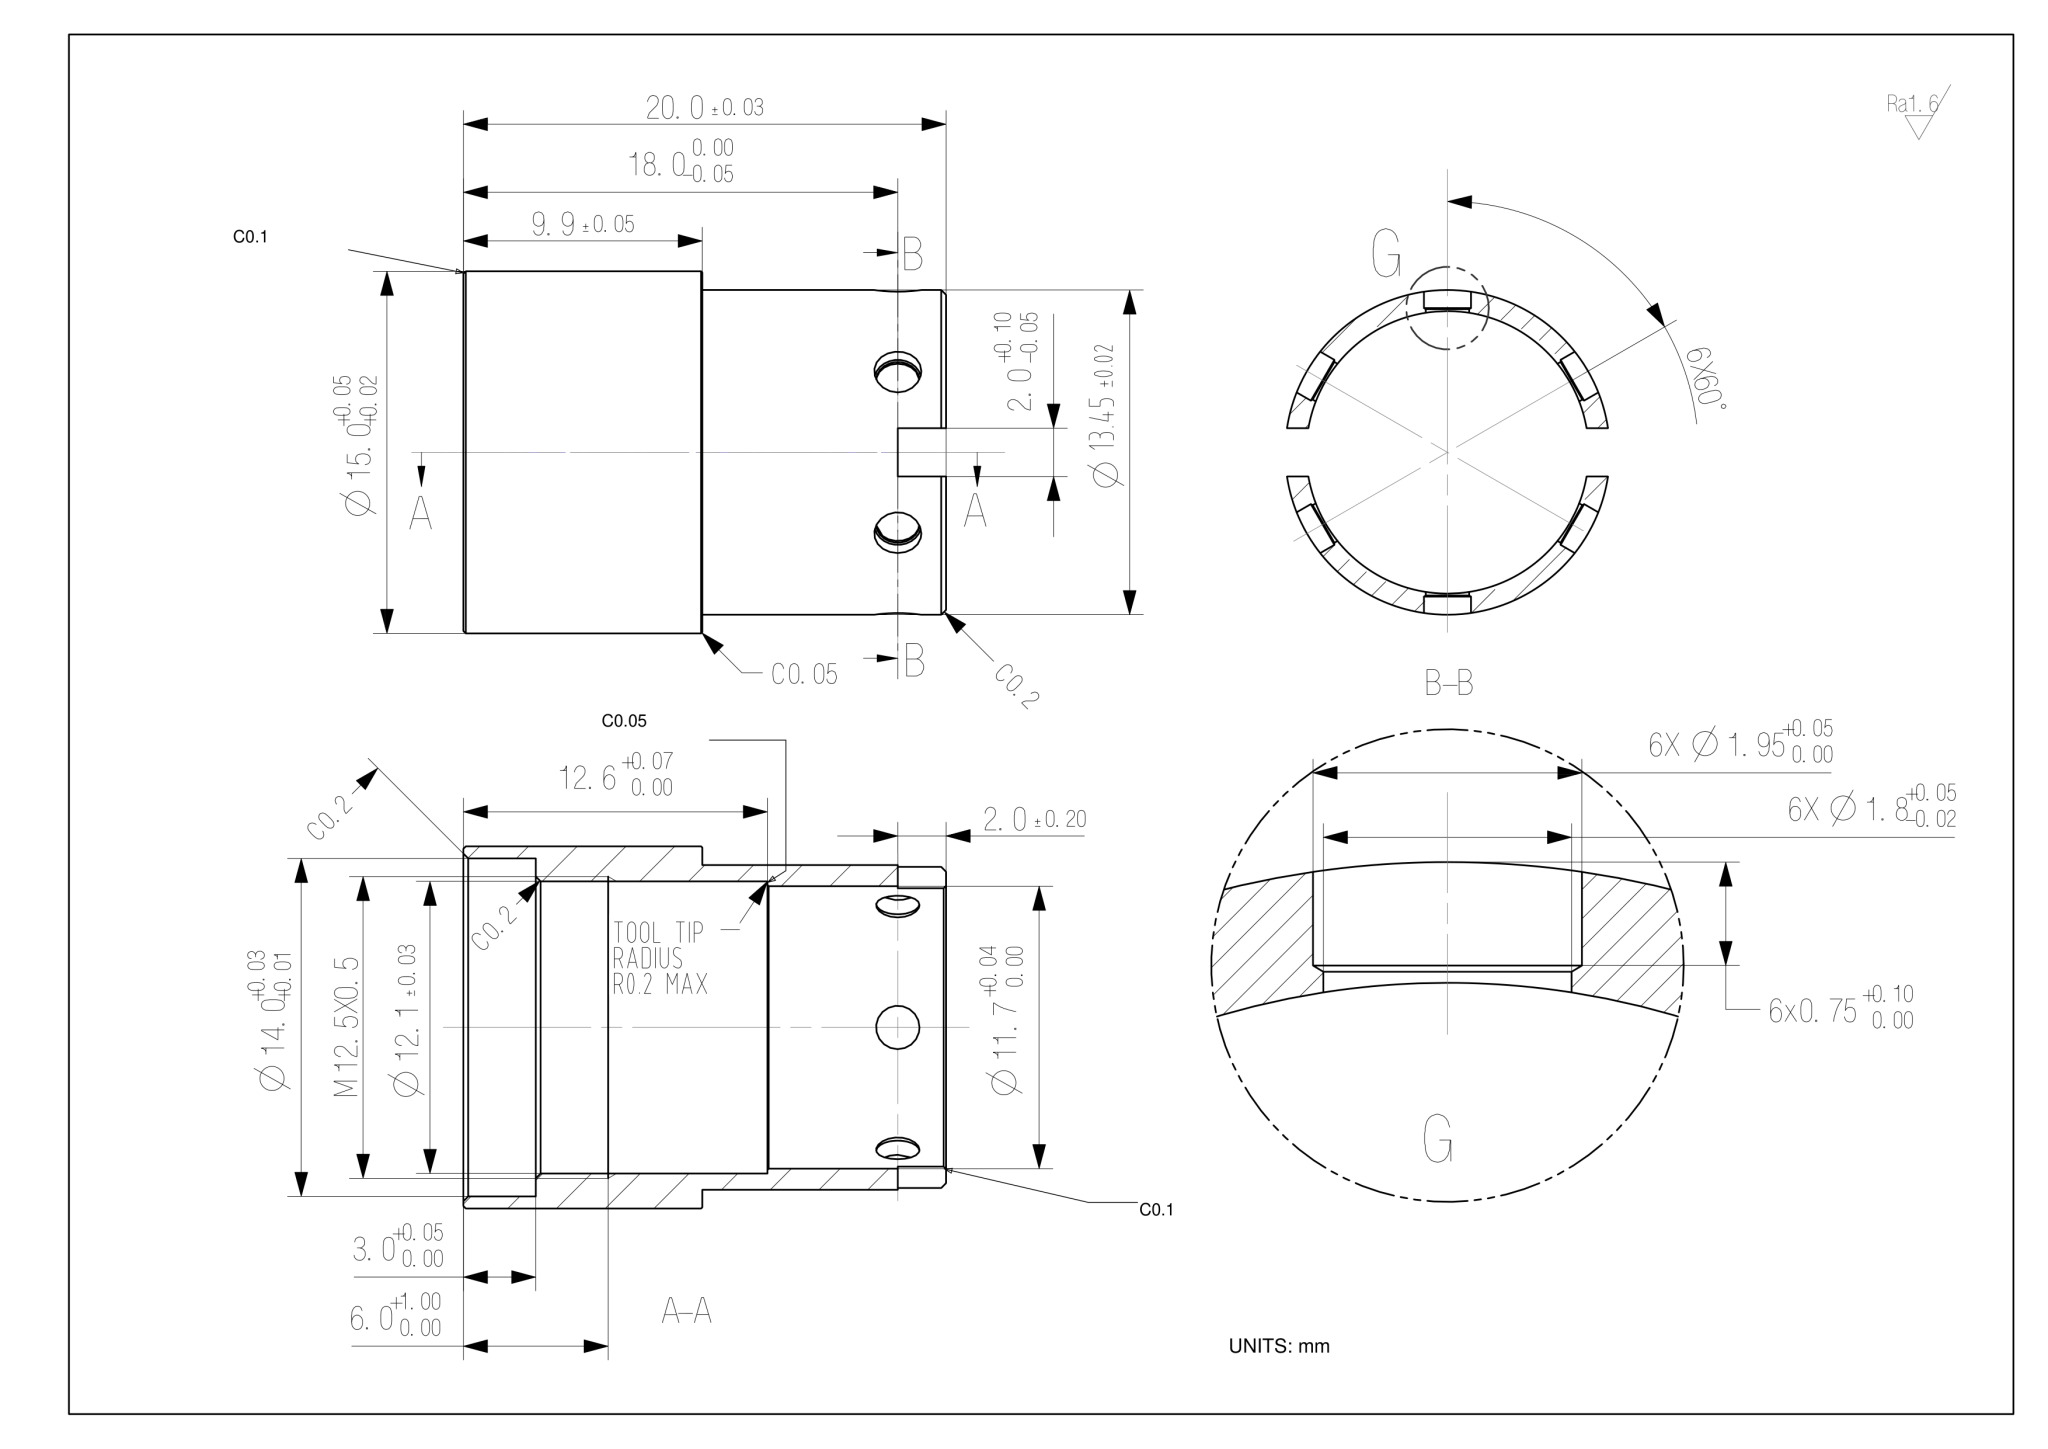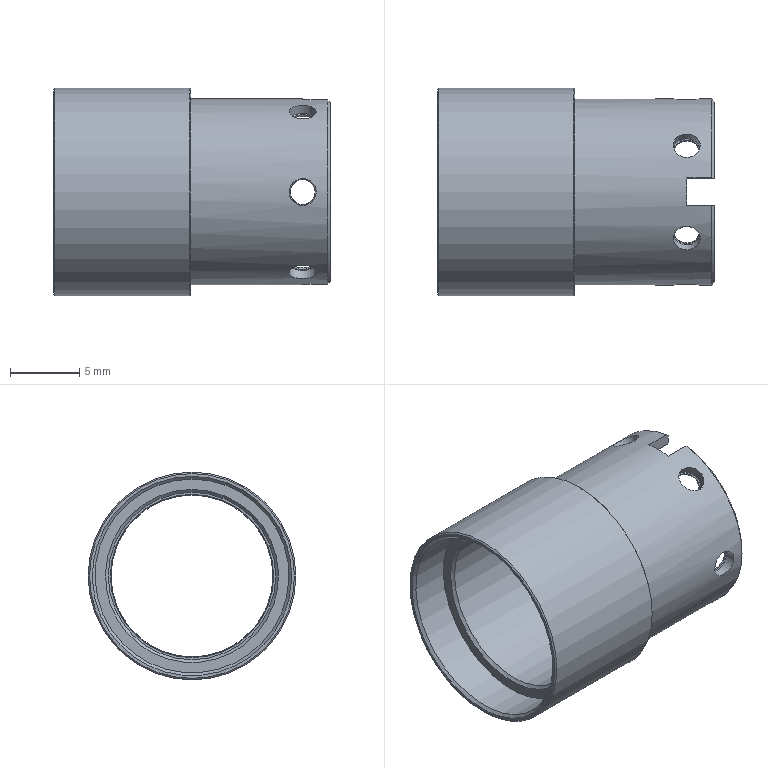Part | NX | mm | 1 solid | 44 faces | box 20 x 15 x 15 mm | volume 798 mm3 | cylinder 17 | cone 15 | plane 12 | commonest cylinder face diameters 1.8 x6 1.95 x6 11.7 x1 12.1 x1 14 x1 15 x1 13.45 x1